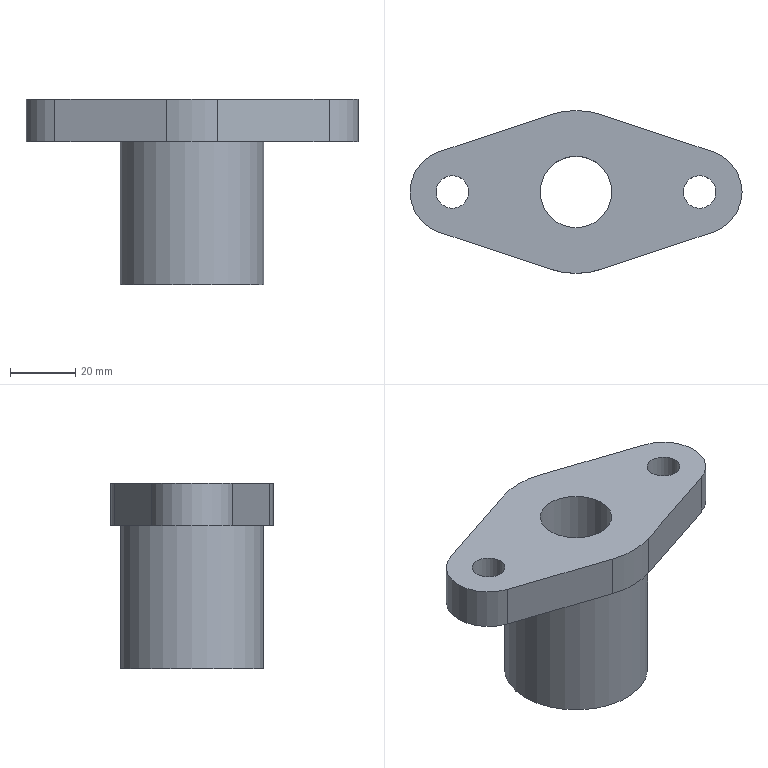Component | NX | 06__GLAND__2 | 1 solid | 15 faces | box 102 x 50 x 57 mm | volume 86309 mm3 | cylinder 8 | plane 6 | cone 1 | commonest cylinder face diameters 26 x2 50 x2 10 x2 22 x1 44 x1
STEP:
#1=CARTESIAN_POINT('',(0.,0.,0.));
#2=DIRECTION('',(0.,0.,1.));
#3=DIRECTION('',(1.,0.,0.));
#4=AXIS2_PLACEMENT_3D('',#1,#2,#3);
#5=CARTESIAN_POINT('',(35.73,-13.604,857.));
#6=VERTEX_POINT('',#5);
#7=CARTESIAN_POINT('',(35.73,11.065,857.));
#8=VERTEX_POINT('',#7);
#9=CARTESIAN_POINT('',(31.625,-1.269,857.));
#10=DIRECTION('',(0.,0.,1.));
#11=DIRECTION('',(-1.,-0.,0.));
#12=AXIS2_PLACEMENT_3D('',#9,#10,#11);
#13=CIRCLE('',#12,13.);
#14=CARTESIAN_POINT('',(31.625,-1.269,870.));
#15=DIRECTION('',(0.,0.,-1.));
#16=DIRECTION('',(1.,0.,0.));
#17=AXIS2_PLACEMENT_3D('',#14,#15,#16);
#18=CYLINDRICAL_SURFACE('',#17,13.);
#19=CARTESIAN_POINT('',(3.142,13.));
#20=DIRECTION('',(-1.,0.));
#21=VECTOR('',#20,1.);
#22=LINE('',#19,#21);
#23=(GEOMETRIC_REPRESENTATION_CONTEXT(2)PARAMETRIC_REPRESENTATION_CONTEXT()REPRESENTATION_CONTEXT('',''));
#24=DEFINITIONAL_REPRESENTATION('',(#22),#23);
#25=PCURVE('',#18,#24);
#26=CARTESIAN_POINT('',(31.625,-1.269,857.));
#27=DIRECTION('',(0.,0.,1.));
#28=DIRECTION('',(-1.,-0.,0.));
#29=AXIS2_PLACEMENT_3D('',#26,#27,#28);
#30=PLANE('',#29);
#31=CARTESIAN_POINT('',(0.,0.));
#32=DIRECTION('',(1.,0.));
#33=AXIS2_PLACEMENT_2D('',#31,#32);
#34=CIRCLE('',#33,13.);
#35=(GEOMETRIC_REPRESENTATION_CONTEXT(2)PARAMETRIC_REPRESENTATION_CONTEXT()REPRESENTATION_CONTEXT('',''));
#36=DEFINITIONAL_REPRESENTATION('',(#34),#35);
#37=PCURVE('',#30,#36);
#38=SURFACE_CURVE('',#13,(#25,#37),.PCURVE_S1.);
#39=EDGE_CURVE('',#6,#8,#38,.T.);
#40=ORIENTED_EDGE('',*,*,#39,.T.);
#41=CARTESIAN_POINT('',(35.73,11.065,870.));
#42=VERTEX_POINT('',#41);
#43=CARTESIAN_POINT('',(35.73,11.065,870.));
#44=DIRECTION('',(0.,0.,-1.));
#45=VECTOR('',#44,1.);
#46=LINE('',#43,#45);
#47=CARTESIAN_POINT('',(-1.25,0.));
#48=DIRECTION('',(0.,1.));
#49=VECTOR('',#48,1.);
#50=LINE('',#47,#49);
#51=(GEOMETRIC_REPRESENTATION_CONTEXT(2)PARAMETRIC_REPRESENTATION_CONTEXT()REPRESENTATION_CONTEXT('',''));
#52=DEFINITIONAL_REPRESENTATION('',(#50),#51);
#53=PCURVE('',#18,#52);
#54=CARTESIAN_POINT('',(35.73,11.065,870.));
#55=DIRECTION('',(-0.3158,-0.9488,0.));
#56=DIRECTION('',(0.9488,-0.3158,0.));
#57=AXIS2_PLACEMENT_3D('',#54,#55,#56);
#58=PLANE('',#57);
#59=CARTESIAN_POINT('',(-0.,0.));
#60=DIRECTION('',(0.,-1.));
#61=VECTOR('',#60,1.);
#62=LINE('',#59,#61);
#63=(GEOMETRIC_REPRESENTATION_CONTEXT(2)PARAMETRIC_REPRESENTATION_CONTEXT()REPRESENTATION_CONTEXT('',''));
#64=DEFINITIONAL_REPRESENTATION('',(#62),#63);
#65=PCURVE('',#58,#64);
#66=SURFACE_CURVE('',#46,(#53,#65),.PCURVE_S1.);
#67=EDGE_CURVE('',#42,#8,#66,.T.);
#68=ORIENTED_EDGE('',*,*,#67,.F.);
#69=CARTESIAN_POINT('',(35.73,-13.604,870.));
#70=VERTEX_POINT('',#69);
#71=CARTESIAN_POINT('',(31.625,-1.269,870.));
#72=DIRECTION('',(0.,0.,1.));
#73=DIRECTION('',(-1.,-0.,0.));
#74=AXIS2_PLACEMENT_3D('',#71,#72,#73);
#75=CIRCLE('',#74,13.);
#76=CARTESIAN_POINT('',(3.142,0.));
#77=DIRECTION('',(-1.,0.));
#78=VECTOR('',#77,1.);
#79=LINE('',#76,#78);
#80=(GEOMETRIC_REPRESENTATION_CONTEXT(2)PARAMETRIC_REPRESENTATION_CONTEXT()REPRESENTATION_CONTEXT('',''));
#81=DEFINITIONAL_REPRESENTATION('',(#79),#80);
#82=PCURVE('',#18,#81);
#83=CARTESIAN_POINT('',(31.625,-1.269,870.));
#84=DIRECTION('',(0.,0.,1.));
#85=DIRECTION('',(-1.,-0.,0.));
#86=AXIS2_PLACEMENT_3D('',#83,#84,#85);
#87=PLANE('',#86);
#88=CARTESIAN_POINT('',(0.,0.));
#89=DIRECTION('',(1.,0.));
#90=AXIS2_PLACEMENT_2D('',#88,#89);
#91=CIRCLE('',#90,13.);
#92=(GEOMETRIC_REPRESENTATION_CONTEXT(2)PARAMETRIC_REPRESENTATION_CONTEXT()REPRESENTATION_CONTEXT('',''));
#93=DEFINITIONAL_REPRESENTATION('',(#91),#92);
#94=PCURVE('',#87,#93);
#95=SURFACE_CURVE('',#75,(#82,#94),.PCURVE_S1.);
#96=EDGE_CURVE('',#70,#42,#95,.T.);
#97=ORIENTED_EDGE('',*,*,#96,.F.);
#98=CARTESIAN_POINT('',(35.73,-13.604,870.));
#99=DIRECTION('',(0.,0.,-1.));
#100=VECTOR('',#99,1.);
#101=LINE('',#98,#100);
#102=CARTESIAN_POINT('',(1.25,0.));
#103=DIRECTION('',(0.,1.));
#104=VECTOR('',#103,1.);
#105=LINE('',#102,#104);
#106=(GEOMETRIC_REPRESENTATION_CONTEXT(2)PARAMETRIC_REPRESENTATION_CONTEXT()REPRESENTATION_CONTEXT('',''));
#107=DEFINITIONAL_REPRESENTATION('',(#105),#106);
#108=PCURVE('',#18,#107);
#109=CARTESIAN_POINT('',(1.52,-24.99,870.));
#110=DIRECTION('',(-0.3158,0.9488,0.));
#111=DIRECTION('',(-0.9488,-0.3158,0.));
#112=AXIS2_PLACEMENT_3D('',#109,#110,#111);
#113=PLANE('',#112);
#114=CARTESIAN_POINT('',(-36.056,0.));
#115=DIRECTION('',(0.,-1.));
#116=VECTOR('',#115,1.);
#117=LINE('',#114,#116);
#118=(GEOMETRIC_REPRESENTATION_CONTEXT(2)PARAMETRIC_REPRESENTATION_CONTEXT()REPRESENTATION_CONTEXT('',''));
#119=DEFINITIONAL_REPRESENTATION('',(#117),#118);
#120=PCURVE('',#113,#119);
#121=SURFACE_CURVE('',#101,(#108,#120),.PCURVE_S1.);
#122=EDGE_CURVE('',#70,#6,#121,.T.);
#123=ORIENTED_EDGE('',*,*,#122,.T.);
#124=EDGE_LOOP('',(#40,#68,#97,#123));
#125=FACE_BOUND('',#124,.T.);
#126=ADVANCED_FACE('',(#125),#18,.T.);
#127=CARTESIAN_POINT('',(1.52,22.451,857.));
#128=VERTEX_POINT('',#127);
#129=CARTESIAN_POINT('',(35.73,11.065,857.));
#130=DIRECTION('',(-0.9488,0.3158,0.));
#131=VECTOR('',#130,1.);
#132=LINE('',#129,#131);
#133=CARTESIAN_POINT('',(0.,-13.));
#134=DIRECTION('',(-1.,0.));
#135=VECTOR('',#134,1.);
#136=LINE('',#133,#135);
#137=(GEOMETRIC_REPRESENTATION_CONTEXT(2)PARAMETRIC_REPRESENTATION_CONTEXT()REPRESENTATION_CONTEXT('',''));
#138=DEFINITIONAL_REPRESENTATION('',(#136),#137);
#139=PCURVE('',#58,#138);
#140=CARTESIAN_POINT('',(-4.105,-12.335));
#141=DIRECTION('',(0.9488,-0.3158));
#142=VECTOR('',#141,1.);
#143=LINE('',#140,#142);
#144=(GEOMETRIC_REPRESENTATION_CONTEXT(2)PARAMETRIC_REPRESENTATION_CONTEXT()REPRESENTATION_CONTEXT('',''));
#145=DEFINITIONAL_REPRESENTATION('',(#143),#144);
#146=PCURVE('',#30,#145);
#147=SURFACE_CURVE('',#132,(#139,#146),.PCURVE_S1.);
#148=EDGE_CURVE('',#8,#128,#147,.T.);
#149=ORIENTED_EDGE('',*,*,#148,.T.);
#150=CARTESIAN_POINT('',(1.52,22.451,870.));
#151=VERTEX_POINT('',#150);
#152=CARTESIAN_POINT('',(1.52,22.451,870.));
#153=DIRECTION('',(0.,0.,-1.));
#154=VECTOR('',#153,1.);
#155=LINE('',#152,#154);
#156=CARTESIAN_POINT('',(-36.056,0.));
#157=DIRECTION('',(0.,-1.));
#158=VECTOR('',#157,1.);
#159=LINE('',#156,#158);
#160=(GEOMETRIC_REPRESENTATION_CONTEXT(2)PARAMETRIC_REPRESENTATION_CONTEXT()REPRESENTATION_CONTEXT('',''));
#161=DEFINITIONAL_REPRESENTATION('',(#159),#160);
#162=PCURVE('',#58,#161);
#163=CARTESIAN_POINT('',(-6.375,-1.269,870.));
#164=DIRECTION('',(0.,0.,-1.));
#165=DIRECTION('',(1.,0.,0.));
#166=AXIS2_PLACEMENT_3D('',#163,#164,#165);
#167=CYLINDRICAL_SURFACE('',#166,25.);
#168=CARTESIAN_POINT('',(5.034,0.));
#169=DIRECTION('',(0.,1.));
#170=VECTOR('',#169,1.);
#171=LINE('',#168,#170);
#172=(GEOMETRIC_REPRESENTATION_CONTEXT(2)PARAMETRIC_REPRESENTATION_CONTEXT()REPRESENTATION_CONTEXT('',''));
#173=DEFINITIONAL_REPRESENTATION('',(#171),#172);
#174=PCURVE('',#167,#173);
#175=SURFACE_CURVE('',#155,(#162,#174),.PCURVE_S1.);
#176=EDGE_CURVE('',#151,#128,#175,.T.);
#177=ORIENTED_EDGE('',*,*,#176,.F.);
#178=CARTESIAN_POINT('',(35.73,11.065,870.));
#179=DIRECTION('',(-0.9488,0.3158,0.));
#180=VECTOR('',#179,1.);
#181=LINE('',#178,#180);
#182=CARTESIAN_POINT('',(0.,0.));
#183=DIRECTION('',(-1.,0.));
#184=VECTOR('',#183,1.);
#185=LINE('',#182,#184);
#186=(GEOMETRIC_REPRESENTATION_CONTEXT(2)PARAMETRIC_REPRESENTATION_CONTEXT()REPRESENTATION_CONTEXT('',''));
#187=DEFINITIONAL_REPRESENTATION('',(#185),#186);
#188=PCURVE('',#58,#187);
#189=CARTESIAN_POINT('',(-4.105,-12.335));
#190=DIRECTION('',(0.9488,-0.3158));
#191=VECTOR('',#190,1.);
#192=LINE('',#189,#191);
#193=(GEOMETRIC_REPRESENTATION_CONTEXT(2)PARAMETRIC_REPRESENTATION_CONTEXT()REPRESENTATION_CONTEXT('',''));
#194=DEFINITIONAL_REPRESENTATION('',(#192),#193);
#195=PCURVE('',#87,#194);
#196=SURFACE_CURVE('',#181,(#188,#195),.PCURVE_S1.);
#197=EDGE_CURVE('',#42,#151,#196,.T.);
#198=ORIENTED_EDGE('',*,*,#197,.F.);
#199=ORIENTED_EDGE('',*,*,#67,.T.);
#200=EDGE_LOOP('',(#149,#177,#198,#199));
#201=FACE_BOUND('',#200,.T.);
#202=ADVANCED_FACE('',(#201),#58,.F.);
#203=CARTESIAN_POINT('',(-14.27,22.451,857.));
#204=VERTEX_POINT('',#203);
#205=CARTESIAN_POINT('',(-6.375,-1.269,857.));
#206=DIRECTION('',(0.,0.,1.));
#207=DIRECTION('',(-1.,-0.,0.));
#208=AXIS2_PLACEMENT_3D('',#205,#206,#207);
#209=CIRCLE('',#208,25.);
#210=CARTESIAN_POINT('',(9.425,13.));
#211=DIRECTION('',(-1.,0.));
#212=VECTOR('',#211,1.);
#213=LINE('',#210,#212);
#214=(GEOMETRIC_REPRESENTATION_CONTEXT(2)PARAMETRIC_REPRESENTATION_CONTEXT()REPRESENTATION_CONTEXT('',''));
#215=DEFINITIONAL_REPRESENTATION('',(#213),#214);
#216=PCURVE('',#167,#215);
#217=CARTESIAN_POINT('',(38.,0.));
#218=DIRECTION('',(1.,-0.));
#219=AXIS2_PLACEMENT_2D('',#217,#218);
#220=CIRCLE('',#219,25.);
#221=(GEOMETRIC_REPRESENTATION_CONTEXT(2)PARAMETRIC_REPRESENTATION_CONTEXT()REPRESENTATION_CONTEXT('',''));
#222=DEFINITIONAL_REPRESENTATION('',(#220),#221);
#223=PCURVE('',#30,#222);
#224=SURFACE_CURVE('',#209,(#216,#223),.PCURVE_S1.);
#225=EDGE_CURVE('',#128,#204,#224,.T.);
#226=ORIENTED_EDGE('',*,*,#225,.T.);
#227=CARTESIAN_POINT('',(-14.27,22.451,870.));
#228=VERTEX_POINT('',#227);
#229=CARTESIAN_POINT('',(-14.27,22.451,870.));
#230=DIRECTION('',(0.,0.,-1.));
#231=VECTOR('',#230,1.);
#232=LINE('',#229,#231);
#233=CARTESIAN_POINT('',(4.391,0.));
#234=DIRECTION('',(0.,1.));
#235=VECTOR('',#234,1.);
#236=LINE('',#233,#235);
#237=(GEOMETRIC_REPRESENTATION_CONTEXT(2)PARAMETRIC_REPRESENTATION_CONTEXT()REPRESENTATION_CONTEXT('',''));
#238=DEFINITIONAL_REPRESENTATION('',(#236),#237);
#239=PCURVE('',#167,#238);
#240=CARTESIAN_POINT('',(-14.27,22.451,870.));
#241=DIRECTION('',(0.3158,-0.9488,0.));
#242=DIRECTION('',(0.9488,0.3158,0.));
#243=AXIS2_PLACEMENT_3D('',#240,#241,#242);
#244=PLANE('',#243);
#245=CARTESIAN_POINT('',(0.,0.));
#246=DIRECTION('',(0.,-1.));
#247=VECTOR('',#246,1.);
#248=LINE('',#245,#247);
#249=(GEOMETRIC_REPRESENTATION_CONTEXT(2)PARAMETRIC_REPRESENTATION_CONTEXT()REPRESENTATION_CONTEXT('',''));
#250=DEFINITIONAL_REPRESENTATION('',(#248),#249);
#251=PCURVE('',#244,#250);
#252=SURFACE_CURVE('',#232,(#239,#251),.PCURVE_S1.);
#253=EDGE_CURVE('',#228,#204,#252,.T.);
#254=ORIENTED_EDGE('',*,*,#253,.F.);
#255=CARTESIAN_POINT('',(-6.375,-1.269,870.));
#256=DIRECTION('',(0.,0.,1.));
#257=DIRECTION('',(-1.,-0.,0.));
#258=AXIS2_PLACEMENT_3D('',#255,#256,#257);
#259=CIRCLE('',#258,25.);
#260=CARTESIAN_POINT('',(9.425,0.));
#261=DIRECTION('',(-1.,0.));
#262=VECTOR('',#261,1.);
#263=LINE('',#260,#262);
#264=(GEOMETRIC_REPRESENTATION_CONTEXT(2)PARAMETRIC_REPRESENTATION_CONTEXT()REPRESENTATION_CONTEXT('',''));
#265=DEFINITIONAL_REPRESENTATION('',(#263),#264);
#266=PCURVE('',#167,#265);
#267=CARTESIAN_POINT('',(38.,0.));
#268=DIRECTION('',(1.,-0.));
#269=AXIS2_PLACEMENT_2D('',#267,#268);
#270=CIRCLE('',#269,25.);
#271=(GEOMETRIC_REPRESENTATION_CONTEXT(2)PARAMETRIC_REPRESENTATION_CONTEXT()REPRESENTATION_CONTEXT('',''));
#272=DEFINITIONAL_REPRESENTATION('',(#270),#271);
#273=PCURVE('',#87,#272);
#274=SURFACE_CURVE('',#259,(#266,#273),.PCURVE_S1.);
#275=EDGE_CURVE('',#151,#228,#274,.T.);
#276=ORIENTED_EDGE('',*,*,#275,.F.);
#277=ORIENTED_EDGE('',*,*,#176,.T.);
#278=EDGE_LOOP('',(#226,#254,#276,#277));
#279=FACE_BOUND('',#278,.T.);
#280=ADVANCED_FACE('',(#279),#167,.T.);
#281=CARTESIAN_POINT('',(-48.48,11.065,857.));
#282=VERTEX_POINT('',#281);
#283=CARTESIAN_POINT('',(-14.27,22.451,857.));
#284=DIRECTION('',(-0.9488,-0.3158,0.));
#285=VECTOR('',#284,1.);
#286=LINE('',#283,#285);
#287=CARTESIAN_POINT('',(0.,-13.));
#288=DIRECTION('',(-1.,0.));
#289=VECTOR('',#288,1.);
#290=LINE('',#287,#289);
#291=(GEOMETRIC_REPRESENTATION_CONTEXT(2)PARAMETRIC_REPRESENTATION_CONTEXT()REPRESENTATION_CONTEXT('',''));
#292=DEFINITIONAL_REPRESENTATION('',(#290),#291);
#293=PCURVE('',#244,#292);
#294=CARTESIAN_POINT('',(45.895,-23.721));
#295=DIRECTION('',(0.9488,0.3158));
#296=VECTOR('',#295,1.);
#297=LINE('',#294,#296);
#298=(GEOMETRIC_REPRESENTATION_CONTEXT(2)PARAMETRIC_REPRESENTATION_CONTEXT()REPRESENTATION_CONTEXT('',''));
#299=DEFINITIONAL_REPRESENTATION('',(#297),#298);
#300=PCURVE('',#30,#299);
#301=SURFACE_CURVE('',#286,(#293,#300),.PCURVE_S1.);
#302=EDGE_CURVE('',#204,#282,#301,.T.);
#303=ORIENTED_EDGE('',*,*,#302,.T.);
#304=CARTESIAN_POINT('',(-48.48,11.065,870.));
#305=VERTEX_POINT('',#304);
#306=CARTESIAN_POINT('',(-48.48,11.065,870.));
#307=DIRECTION('',(0.,0.,-1.));
#308=VECTOR('',#307,1.);
#309=LINE('',#306,#308);
#310=CARTESIAN_POINT('',(-36.056,0.));
#311=DIRECTION('',(0.,-1.));
#312=VECTOR('',#311,1.);
#313=LINE('',#310,#312);
#314=(GEOMETRIC_REPRESENTATION_CONTEXT(2)PARAMETRIC_REPRESENTATION_CONTEXT()REPRESENTATION_CONTEXT('',''));
#315=DEFINITIONAL_REPRESENTATION('',(#313),#314);
#316=PCURVE('',#244,#315);
#317=CARTESIAN_POINT('',(-44.375,-1.269,870.));
#318=DIRECTION('',(0.,0.,-1.));
#319=DIRECTION('',(1.,0.,0.));
#320=AXIS2_PLACEMENT_3D('',#317,#318,#319);
#321=CYLINDRICAL_SURFACE('',#320,13.);
#322=CARTESIAN_POINT('',(4.391,0.));
#323=DIRECTION('',(0.,1.));
#324=VECTOR('',#323,1.);
#325=LINE('',#322,#324);
#326=(GEOMETRIC_REPRESENTATION_CONTEXT(2)PARAMETRIC_REPRESENTATION_CONTEXT()REPRESENTATION_CONTEXT('',''));
#327=DEFINITIONAL_REPRESENTATION('',(#325),#326);
#328=PCURVE('',#321,#327);
#329=SURFACE_CURVE('',#309,(#316,#328),.PCURVE_S1.);
#330=EDGE_CURVE('',#305,#282,#329,.T.);
#331=ORIENTED_EDGE('',*,*,#330,.F.);
#332=CARTESIAN_POINT('',(-14.27,22.451,870.));
#333=DIRECTION('',(-0.9488,-0.3158,0.));
#334=VECTOR('',#333,1.);
#335=LINE('',#332,#334);
#336=CARTESIAN_POINT('',(0.,0.));
#337=DIRECTION('',(-1.,0.));
#338=VECTOR('',#337,1.);
#339=LINE('',#336,#338);
#340=(GEOMETRIC_REPRESENTATION_CONTEXT(2)PARAMETRIC_REPRESENTATION_CONTEXT()REPRESENTATION_CONTEXT('',''));
#341=DEFINITIONAL_REPRESENTATION('',(#339),#340);
#342=PCURVE('',#244,#341);
#343=CARTESIAN_POINT('',(45.895,-23.721));
#344=DIRECTION('',(0.9488,0.3158));
#345=VECTOR('',#344,1.);
#346=LINE('',#343,#345);
#347=(GEOMETRIC_REPRESENTATION_CONTEXT(2)PARAMETRIC_REPRESENTATION_CONTEXT()REPRESENTATION_CONTEXT('',''));
#348=DEFINITIONAL_REPRESENTATION('',(#346),#347);
#349=PCURVE('',#87,#348);
#350=SURFACE_CURVE('',#335,(#342,#349),.PCURVE_S1.);
#351=EDGE_CURVE('',#228,#305,#350,.T.);
#352=ORIENTED_EDGE('',*,*,#351,.F.);
#353=ORIENTED_EDGE('',*,*,#253,.T.);
#354=EDGE_LOOP('',(#303,#331,#352,#353));
#355=FACE_BOUND('',#354,.T.);
#356=ADVANCED_FACE('',(#355),#244,.F.);
#357=CARTESIAN_POINT('',(-48.48,-13.604,857.));
#358=VERTEX_POINT('',#357);
#359=CARTESIAN_POINT('',(-44.375,-1.269,857.));
#360=DIRECTION('',(0.,0.,1.));
#361=DIRECTION('',(1.,0.,0.));
#362=AXIS2_PLACEMENT_3D('',#359,#360,#361);
#363=CIRCLE('',#362,13.);
#364=CARTESIAN_POINT('',(6.283,13.));
#365=DIRECTION('',(-1.,0.));
#366=VECTOR('',#365,1.);
#367=LINE('',#364,#366);
#368=(GEOMETRIC_REPRESENTATION_CONTEXT(2)PARAMETRIC_REPRESENTATION_CONTEXT()REPRESENTATION_CONTEXT('',''));
#369=DEFINITIONAL_REPRESENTATION('',(#367),#368);
#370=PCURVE('',#321,#369);
#371=CARTESIAN_POINT('',(76.,0.));
#372=DIRECTION('',(-1.,0.));
#373=AXIS2_PLACEMENT_2D('',#371,#372);
#374=CIRCLE('',#373,13.);
#375=(GEOMETRIC_REPRESENTATION_CONTEXT(2)PARAMETRIC_REPRESENTATION_CONTEXT()REPRESENTATION_CONTEXT('',''));
#376=DEFINITIONAL_REPRESENTATION('',(#374),#375);
#377=PCURVE('',#30,#376);
#378=SURFACE_CURVE('',#363,(#370,#377),.PCURVE_S1.);
#379=EDGE_CURVE('',#282,#358,#378,.T.);
#380=ORIENTED_EDGE('',*,*,#379,.T.);
#381=CARTESIAN_POINT('',(-48.48,-13.604,870.));
#382=VERTEX_POINT('',#381);
#383=CARTESIAN_POINT('',(-48.48,-13.604,870.));
#384=DIRECTION('',(0.,0.,-1.));
#385=VECTOR('',#384,1.);
#386=LINE('',#383,#385);
#387=CARTESIAN_POINT('',(1.892,0.));
#388=DIRECTION('',(0.,1.));
#389=VECTOR('',#388,1.);
#390=LINE('',#387,#389);
#391=(GEOMETRIC_REPRESENTATION_CONTEXT(2)PARAMETRIC_REPRESENTATION_CONTEXT()REPRESENTATION_CONTEXT('',''));
#392=DEFINITIONAL_REPRESENTATION('',(#390),#391);
#393=PCURVE('',#321,#392);
#394=CARTESIAN_POINT('',(-48.48,-13.604,870.));
#395=DIRECTION('',(0.3158,0.9488,0.));
#396=DIRECTION('',(-0.9488,0.3158,0.));
#397=AXIS2_PLACEMENT_3D('',#394,#395,#396);
#398=PLANE('',#397);
#399=CARTESIAN_POINT('',(-0.,0.));
#400=DIRECTION('',(0.,-1.));
#401=VECTOR('',#400,1.);
#402=LINE('',#399,#401);
#403=(GEOMETRIC_REPRESENTATION_CONTEXT(2)PARAMETRIC_REPRESENTATION_CONTEXT()REPRESENTATION_CONTEXT('',''));
#404=DEFINITIONAL_REPRESENTATION('',(#402),#403);
#405=PCURVE('',#398,#404);
#406=SURFACE_CURVE('',#386,(#393,#405),.PCURVE_S1.);
#407=EDGE_CURVE('',#382,#358,#406,.T.);
#408=ORIENTED_EDGE('',*,*,#407,.F.);
#409=CARTESIAN_POINT('',(-44.375,-1.269,870.));
#410=DIRECTION('',(0.,0.,1.));
#411=DIRECTION('',(1.,0.,0.));
#412=AXIS2_PLACEMENT_3D('',#409,#410,#411);
#413=CIRCLE('',#412,13.);
#414=CARTESIAN_POINT('',(6.283,0.));
#415=DIRECTION('',(-1.,0.));
#416=VECTOR('',#415,1.);
#417=LINE('',#414,#416);
#418=(GEOMETRIC_REPRESENTATION_CONTEXT(2)PARAMETRIC_REPRESENTATION_CONTEXT()REPRESENTATION_CONTEXT('',''));
#419=DEFINITIONAL_REPRESENTATION('',(#417),#418);
#420=PCURVE('',#321,#419);
#421=CARTESIAN_POINT('',(76.,0.));
#422=DIRECTION('',(-1.,0.));
#423=AXIS2_PLACEMENT_2D('',#421,#422);
#424=CIRCLE('',#423,13.);
#425=(GEOMETRIC_REPRESENTATION_CONTEXT(2)PARAMETRIC_REPRESENTATION_CONTEXT()REPRESENTATION_CONTEXT('',''));
#426=DEFINITIONAL_REPRESENTATION('',(#424),#425);
#427=PCURVE('',#87,#426);
#428=SURFACE_CURVE('',#413,(#420,#427),.PCURVE_S1.);
#429=EDGE_CURVE('',#305,#382,#428,.T.);
#430=ORIENTED_EDGE('',*,*,#429,.F.);
#431=ORIENTED_EDGE('',*,*,#330,.T.);
#432=EDGE_LOOP('',(#380,#408,#430,#431));
#433=FACE_BOUND('',#432,.T.);
#434=ADVANCED_FACE('',(#433),#321,.T.);
#435=CARTESIAN_POINT('',(-14.27,-24.99,857.));
#436=VERTEX_POINT('',#435);
#437=CARTESIAN_POINT('',(-48.48,-13.604,857.));
#438=DIRECTION('',(0.9488,-0.3158,0.));
#439=VECTOR('',#438,1.);
#440=LINE('',#437,#439);
#441=CARTESIAN_POINT('',(0.,-13.));
#442=DIRECTION('',(-1.,0.));
#443=VECTOR('',#442,1.);
#444=LINE('',#441,#443);
#445=(GEOMETRIC_REPRESENTATION_CONTEXT(2)PARAMETRIC_REPRESENTATION_CONTEXT()REPRESENTATION_CONTEXT('',''));
#446=DEFINITIONAL_REPRESENTATION('',(#444),#445);
#447=PCURVE('',#398,#446);
#448=CARTESIAN_POINT('',(80.105,12.335));
#449=DIRECTION('',(-0.9488,0.3158));
#450=VECTOR('',#449,1.);
#451=LINE('',#448,#450);
#452=(GEOMETRIC_REPRESENTATION_CONTEXT(2)PARAMETRIC_REPRESENTATION_CONTEXT()REPRESENTATION_CONTEXT('',''));
#453=DEFINITIONAL_REPRESENTATION('',(#451),#452);
#454=PCURVE('',#30,#453);
#455=SURFACE_CURVE('',#440,(#447,#454),.PCURVE_S1.);
#456=EDGE_CURVE('',#358,#436,#455,.T.);
#457=ORIENTED_EDGE('',*,*,#456,.T.);
#458=CARTESIAN_POINT('',(-14.27,-24.99,870.));
#459=VERTEX_POINT('',#458);
#460=CARTESIAN_POINT('',(-14.27,-24.99,870.));
#461=DIRECTION('',(0.,0.,-1.));
#462=VECTOR('',#461,1.);
#463=LINE('',#460,#462);
#464=CARTESIAN_POINT('',(-36.056,0.));
#465=DIRECTION('',(0.,-1.));
#466=VECTOR('',#465,1.);
#467=LINE('',#464,#466);
#468=(GEOMETRIC_REPRESENTATION_CONTEXT(2)PARAMETRIC_REPRESENTATION_CONTEXT()REPRESENTATION_CONTEXT('',''));
#469=DEFINITIONAL_REPRESENTATION('',(#467),#468);
#470=PCURVE('',#398,#469);
#471=CARTESIAN_POINT('',(-6.375,-1.269,870.));
#472=DIRECTION('',(0.,0.,-1.));
#473=DIRECTION('',(1.,0.,0.));
#474=AXIS2_PLACEMENT_3D('',#471,#472,#473);
#475=CYLINDRICAL_SURFACE('',#474,25.);
#476=CARTESIAN_POINT('',(1.892,0.));
#477=DIRECTION('',(0.,1.));
#478=VECTOR('',#477,1.);
#479=LINE('',#476,#478);
#480=(GEOMETRIC_REPRESENTATION_CONTEXT(2)PARAMETRIC_REPRESENTATION_CONTEXT()REPRESENTATION_CONTEXT('',''));
#481=DEFINITIONAL_REPRESENTATION('',(#479),#480);
#482=PCURVE('',#475,#481);
#483=SURFACE_CURVE('',#463,(#470,#482),.PCURVE_S1.);
#484=EDGE_CURVE('',#459,#436,#483,.T.);
#485=ORIENTED_EDGE('',*,*,#484,.F.);
#486=CARTESIAN_POINT('',(-48.48,-13.604,870.));
#487=DIRECTION('',(0.9488,-0.3158,0.));
#488=VECTOR('',#487,1.);
#489=LINE('',#486,#488);
#490=CARTESIAN_POINT('',(0.,0.));
#491=DIRECTION('',(-1.,0.));
#492=VECTOR('',#491,1.);
#493=LINE('',#490,#492);
#494=(GEOMETRIC_REPRESENTATION_CONTEXT(2)PARAMETRIC_REPRESENTATION_CONTEXT()REPRESENTATION_CONTEXT('',''));
#495=DEFINITIONAL_REPRESENTATION('',(#493),#494);
#496=PCURVE('',#398,#495);
#497=CARTESIAN_POINT('',(80.105,12.335));
#498=DIRECTION('',(-0.9488,0.3158));
#499=VECTOR('',#498,1.);
#500=LINE('',#497,#499);
#501=(GEOMETRIC_REPRESENTATION_CONTEXT(2)PARAMETRIC_REPRESENTATION_CONTEXT()REPRESENTATION_CONTEXT('',''));
#502=DEFINITIONAL_REPRESENTATION('',(#500),#501);
#503=PCURVE('',#87,#502);
#504=SURFACE_CURVE('',#489,(#496,#503),.PCURVE_S1.);
#505=EDGE_CURVE('',#382,#459,#504,.T.);
#506=ORIENTED_EDGE('',*,*,#505,.F.);
#507=ORIENTED_EDGE('',*,*,#407,.T.);
#508=EDGE_LOOP('',(#457,#485,#506,#507));
#509=FACE_BOUND('',#508,.T.);
#510=ADVANCED_FACE('',(#509),#398,.F.);
#511=CARTESIAN_POINT('',(1.52,-24.99,857.));
#512=VERTEX_POINT('',#511);
#513=CARTESIAN_POINT('',(-6.375,-1.269,857.));
#514=DIRECTION('',(0.,0.,1.));
#515=DIRECTION('',(-1.,-0.,0.));
#516=AXIS2_PLACEMENT_3D('',#513,#514,#515);
#517=CIRCLE('',#516,25.);
#518=CARTESIAN_POINT('',(3.142,13.));
#519=DIRECTION('',(-1.,0.));
#520=VECTOR('',#519,1.);
#521=LINE('',#518,#520);
#522=(GEOMETRIC_REPRESENTATION_CONTEXT(2)PARAMETRIC_REPRESENTATION_CONTEXT()REPRESENTATION_CONTEXT('',''));
#523=DEFINITIONAL_REPRESENTATION('',(#521),#522);
#524=PCURVE('',#475,#523);
#525=CARTESIAN_POINT('',(38.,0.));
#526=DIRECTION('',(1.,-0.));
#527=AXIS2_PLACEMENT_2D('',#525,#526);
#528=CIRCLE('',#527,25.);
#529=(GEOMETRIC_REPRESENTATION_CONTEXT(2)PARAMETRIC_REPRESENTATION_CONTEXT()REPRESENTATION_CONTEXT('',''));
#530=DEFINITIONAL_REPRESENTATION('',(#528),#529);
#531=PCURVE('',#30,#530);
#532=SURFACE_CURVE('',#517,(#524,#531),.PCURVE_S1.);
#533=EDGE_CURVE('',#436,#512,#532,.T.);
#534=ORIENTED_EDGE('',*,*,#533,.T.);
#535=CARTESIAN_POINT('',(1.52,-24.99,870.));
#536=VERTEX_POINT('',#535);
#537=CARTESIAN_POINT('',(1.52,-24.99,870.));
#538=DIRECTION('',(0.,0.,-1.));
#539=VECTOR('',#538,1.);
#540=LINE('',#537,#539);
#541=CARTESIAN_POINT('',(1.25,0.));
#542=DIRECTION('',(0.,1.));
#543=VECTOR('',#542,1.);
#544=LINE('',#541,#543);
#545=(GEOMETRIC_REPRESENTATION_CONTEXT(2)PARAMETRIC_REPRESENTATION_CONTEXT()REPRESENTATION_CONTEXT('',''));
#546=DEFINITIONAL_REPRESENTATION('',(#544),#545);
#547=PCURVE('',#475,#546);
#548=CARTESIAN_POINT('',(0.,0.));
#549=DIRECTION('',(0.,-1.));
#550=VECTOR('',#549,1.);
#551=LINE('',#548,#550);
#552=(GEOMETRIC_REPRESENTATION_CONTEXT(2)PARAMETRIC_REPRESENTATION_CONTEXT()REPRESENTATION_CONTEXT('',''));
#553=DEFINITIONAL_REPRESENTATION('',(#551),#552);
#554=PCURVE('',#113,#553);
#555=SURFACE_CURVE('',#540,(#547,#554),.PCURVE_S1.);
#556=EDGE_CURVE('',#536,#512,#555,.T.);
#557=ORIENTED_EDGE('',*,*,#556,.F.);
#558=CARTESIAN_POINT('',(-6.375,-1.269,870.));
#559=DIRECTION('',(0.,0.,1.));
#560=DIRECTION('',(-1.,-0.,0.));
#561=AXIS2_PLACEMENT_3D('',#558,#559,#560);
#562=CIRCLE('',#561,25.);
#563=CARTESIAN_POINT('',(3.142,0.));
#564=DIRECTION('',(-1.,0.));
#565=VECTOR('',#564,1.);
#566=LINE('',#563,#565);
#567=(GEOMETRIC_REPRESENTATION_CONTEXT(2)PARAMETRIC_REPRESENTATION_CONTEXT()REPRESENTATION_CONTEXT('',''));
#568=DEFINITIONAL_REPRESENTATION('',(#566),#567);
#569=PCURVE('',#475,#568);
#570=CARTESIAN_POINT('',(38.,0.));
#571=DIRECTION('',(1.,-0.));
#572=AXIS2_PLACEMENT_2D('',#570,#571);
#573=CIRCLE('',#572,25.);
#574=(GEOMETRIC_REPRESENTATION_CONTEXT(2)PARAMETRIC_REPRESENTATION_CONTEXT()REPRESENTATION_CONTEXT('',''));
#575=DEFINITIONAL_REPRESENTATION('',(#573),#574);
#576=PCURVE('',#87,#575);
#577=SURFACE_CURVE('',#562,(#569,#576),.PCURVE_S1.);
#578=EDGE_CURVE('',#459,#536,#577,.T.);
#579=ORIENTED_EDGE('',*,*,#578,.F.);
#580=ORIENTED_EDGE('',*,*,#484,.T.);
#581=EDGE_LOOP('',(#534,#557,#579,#580));
#582=FACE_BOUND('',#581,.T.);
#583=ADVANCED_FACE('',(#582),#475,.T.);
#584=CARTESIAN_POINT('',(-17.375,-1.269,819.351));
#585=VERTEX_POINT('',#584);
#586=CARTESIAN_POINT('',(-6.375,-1.269,819.351));
#587=DIRECTION('',(0.,0.,-1.));
#588=DIRECTION('',(-1.,-0.,0.));
#589=AXIS2_PLACEMENT_3D('',#586,#587,#588);
#590=CIRCLE('',#589,11.);
#591=CARTESIAN_POINT('',(-6.375,-1.269,870.));
#592=DIRECTION('',(0.,0.,-1.));
#593=DIRECTION('',(1.,0.,0.));
#594=AXIS2_PLACEMENT_3D('',#591,#592,#593);
#595=CYLINDRICAL_SURFACE('',#594,11.);
#596=CARTESIAN_POINT('',(3.142,50.649));
#597=DIRECTION('',(1.,0.));
#598=VECTOR('',#597,1.);
#599=LINE('',#596,#598);
#600=(GEOMETRIC_REPRESENTATION_CONTEXT(2)PARAMETRIC_REPRESENTATION_CONTEXT()REPRESENTATION_CONTEXT('',''));
#601=DEFINITIONAL_REPRESENTATION('',(#599),#600);
#602=PCURVE('',#595,#601);
#603=CARTESIAN_POINT('',(-6.375,-1.269,813.));
#604=DIRECTION('',(0.,0.,-1.));
#605=DIRECTION('',(1.,0.,0.));
#606=AXIS2_PLACEMENT_3D('',#603,#604,#605);
#607=CONICAL_SURFACE('',#606,22.,1.047);
#608=CARTESIAN_POINT('',(3.142,-6.351));
#609=DIRECTION('',(1.,0.));
#610=VECTOR('',#609,1.);
#611=LINE('',#608,#610);
#612=(GEOMETRIC_REPRESENTATION_CONTEXT(2)PARAMETRIC_REPRESENTATION_CONTEXT()REPRESENTATION_CONTEXT('',''));
#613=DEFINITIONAL_REPRESENTATION('',(#611),#612);
#614=PCURVE('',#607,#613);
#615=SURFACE_CURVE('',#590,(#602,#614),.PCURVE_S1.);
#616=EDGE_CURVE('',#585,#585,#615,.T.);
#617=ORIENTED_EDGE('',*,*,#616,.F.);
#618=CARTESIAN_POINT('',(-17.375,-1.269,870.));
#619=VERTEX_POINT('',#618);
#620=CARTESIAN_POINT('',(-17.375,-1.269,870.));
#621=CARTESIAN_POINT('',(-17.375,-1.269,819.351));
#622=B_SPLINE_CURVE_WITH_KNOTS('',1,(#620,#621),.UNSPECIFIED.,.F.,.F.,(2,2),(0.,50.649),.PIECEWISE_BEZIER_KNOTS.);
#623=CARTESIAN_POINT('',(3.142,0.));
#624=DIRECTION('',(0.,1.));
#625=VECTOR('',#624,1.);
#626=LINE('',#623,#625);
#627=(GEOMETRIC_REPRESENTATION_CONTEXT(2)PARAMETRIC_REPRESENTATION_CONTEXT()REPRESENTATION_CONTEXT('',''));
#628=DEFINITIONAL_REPRESENTATION('',(#626),#627);
#629=PCURVE('',#595,#628);
#630=CARTESIAN_POINT('',(9.425,0.));
#631=DIRECTION('',(0.,1.));
#632=VECTOR('',#631,1.);
#633=LINE('',#630,#632);
#634=(GEOMETRIC_REPRESENTATION_CONTEXT(2)PARAMETRIC_REPRESENTATION_CONTEXT()REPRESENTATION_CONTEXT('',''));
#635=DEFINITIONAL_REPRESENTATION('',(#633),#634);
#636=PCURVE('',#595,#635);
#637=SEAM_CURVE('',#622,(#629,#636),.PCURVE_S1.);
#638=EDGE_CURVE('',#619,#585,#637,.T.);
#639=ORIENTED_EDGE('',*,*,#638,.F.);
#640=CARTESIAN_POINT('',(-6.375,-1.269,870.));
#641=DIRECTION('',(0.,0.,1.));
#642=DIRECTION('',(-1.,-0.,0.));
#643=AXIS2_PLACEMENT_3D('',#640,#641,#642);
#644=CIRCLE('',#643,11.);
#645=CARTESIAN_POINT('',(9.425,0.));
#646=DIRECTION('',(-1.,0.));
#647=VECTOR('',#646,1.);
#648=LINE('',#645,#647);
#649=(GEOMETRIC_REPRESENTATION_CONTEXT(2)PARAMETRIC_REPRESENTATION_CONTEXT()REPRESENTATION_CONTEXT('',''));
#650=DEFINITIONAL_REPRESENTATION('',(#648),#649);
#651=PCURVE('',#595,#650);
#652=CARTESIAN_POINT('',(38.,0.));
#653=DIRECTION('',(1.,-0.));
#654=AXIS2_PLACEMENT_2D('',#652,#653);
#655=CIRCLE('',#654,11.);
#656=(GEOMETRIC_REPRESENTATION_CONTEXT(2)PARAMETRIC_REPRESENTATION_CONTEXT()REPRESENTATION_CONTEXT('',''));
#657=DEFINITIONAL_REPRESENTATION('',(#655),#656);
#658=PCURVE('',#87,#657);
#659=SURFACE_CURVE('',#644,(#651,#658),.PCURVE_S1.);
#660=EDGE_CURVE('',#619,#619,#659,.T.);
#661=ORIENTED_EDGE('',*,*,#660,.F.);
#662=ORIENTED_EDGE('',*,*,#638,.T.);
#663=EDGE_LOOP('',(#617,#639,#661,#662));
#664=FACE_BOUND('',#663,.F.);
#665=ADVANCED_FACE('',(#664),#595,.F.);
#666=CARTESIAN_POINT('',(26.625,-1.269,870.));
#667=VERTEX_POINT('',#666);
#668=CARTESIAN_POINT('',(31.625,-1.269,870.));
#669=DIRECTION('',(0.,0.,1.));
#670=DIRECTION('',(-1.,-0.,0.));
#671=AXIS2_PLACEMENT_3D('',#668,#669,#670);
#672=CIRCLE('',#671,5.);
#673=CARTESIAN_POINT('',(31.625,-1.269,870.));
#674=DIRECTION('',(0.,0.,-1.));
#675=DIRECTION('',(1.,0.,0.));
#676=AXIS2_PLACEMENT_3D('',#673,#674,#675);
#677=CYLINDRICAL_SURFACE('',#676,5.);
#678=CARTESIAN_POINT('',(9.425,0.));
#679=DIRECTION('',(-1.,0.));
#680=VECTOR('',#679,1.);
#681=LINE('',#678,#680);
#682=(GEOMETRIC_REPRESENTATION_CONTEXT(2)PARAMETRIC_REPRESENTATION_CONTEXT()REPRESENTATION_CONTEXT('',''));
#683=DEFINITIONAL_REPRESENTATION('',(#681),#682);
#684=PCURVE('',#677,#683);
#685=CARTESIAN_POINT('',(0.,0.));
#686=DIRECTION('',(1.,-0.));
#687=AXIS2_PLACEMENT_2D('',#685,#686);
#688=CIRCLE('',#687,5.);
#689=(GEOMETRIC_REPRESENTATION_CONTEXT(2)PARAMETRIC_REPRESENTATION_CONTEXT()REPRESENTATION_CONTEXT('',''));
#690=DEFINITIONAL_REPRESENTATION('',(#688),#689);
#691=PCURVE('',#87,#690);
#692=SURFACE_CURVE('',#672,(#684,#691),.PCURVE_S1.);
#693=EDGE_CURVE('',#667,#667,#692,.T.);
#694=ORIENTED_EDGE('',*,*,#693,.F.);
#695=CARTESIAN_POINT('',(26.625,-1.269,857.));
#696=VERTEX_POINT('',#695);
#697=CARTESIAN_POINT('',(26.625,-1.269,870.));
#698=CARTESIAN_POINT('',(26.625,-1.269,857.));
#699=B_SPLINE_CURVE_WITH_KNOTS('',1,(#697,#698),.UNSPECIFIED.,.F.,.F.,(2,2),(0.,13.),.PIECEWISE_BEZIER_KNOTS.);
#700=CARTESIAN_POINT('',(9.425,0.));
#701=DIRECTION('',(0.,1.));
#702=VECTOR('',#701,1.);
#703=LINE('',#700,#702);
#704=(GEOMETRIC_REPRESENTATION_CONTEXT(2)PARAMETRIC_REPRESENTATION_CONTEXT()REPRESENTATION_CONTEXT('',''));
#705=DEFINITIONAL_REPRESENTATION('',(#703),#704);
#706=PCURVE('',#677,#705);
#707=CARTESIAN_POINT('',(3.142,0.));
#708=DIRECTION('',(0.,1.));
#709=VECTOR('',#708,1.);
#710=LINE('',#707,#709);
#711=(GEOMETRIC_REPRESENTATION_CONTEXT(2)PARAMETRIC_REPRESENTATION_CONTEXT()REPRESENTATION_CONTEXT('',''));
#712=DEFINITIONAL_REPRESENTATION('',(#710),#711);
#713=PCURVE('',#677,#712);
#714=SEAM_CURVE('',#699,(#706,#713),.PCURVE_S1.);
#715=EDGE_CURVE('',#667,#696,#714,.T.);
#716=ORIENTED_EDGE('',*,*,#715,.T.);
#717=CARTESIAN_POINT('',(31.625,-1.269,857.));
#718=DIRECTION('',(0.,0.,1.));
#719=DIRECTION('',(-1.,-0.,0.));
#720=AXIS2_PLACEMENT_3D('',#717,#718,#719);
#721=CIRCLE('',#720,5.);
#722=CARTESIAN_POINT('',(9.425,13.));
#723=DIRECTION('',(-1.,0.));
#724=VECTOR('',#723,1.);
#725=LINE('',#722,#724);
#726=(GEOMETRIC_REPRESENTATION_CONTEXT(2)PARAMETRIC_REPRESENTATION_CONTEXT()REPRESENTATION_CONTEXT('',''));
#727=DEFINITIONAL_REPRESENTATION('',(#725),#726);
#728=PCURVE('',#677,#727);
#729=CARTESIAN_POINT('',(0.,0.));
#730=DIRECTION('',(1.,-0.));
#731=AXIS2_PLACEMENT_2D('',#729,#730);
#732=CIRCLE('',#731,5.);
#733=(GEOMETRIC_REPRESENTATION_CONTEXT(2)PARAMETRIC_REPRESENTATION_CONTEXT()REPRESENTATION_CONTEXT('',''));
#734=DEFINITIONAL_REPRESENTATION('',(#732),#733);
#735=PCURVE('',#30,#734);
#736=SURFACE_CURVE('',#721,(#728,#735),.PCURVE_S1.);
#737=EDGE_CURVE('',#696,#696,#736,.T.);
#738=ORIENTED_EDGE('',*,*,#737,.T.);
#739=ORIENTED_EDGE('',*,*,#715,.F.);
#740=EDGE_LOOP('',(#694,#716,#738,#739));
#741=FACE_BOUND('',#740,.F.);
#742=ADVANCED_FACE('',(#741),#677,.F.);
#743=CARTESIAN_POINT('',(1.52,-24.99,857.));
#744=DIRECTION('',(0.9488,0.3158,0.));
#745=VECTOR('',#744,1.);
#746=LINE('',#743,#745);
#747=CARTESIAN_POINT('',(0.,-13.));
#748=DIRECTION('',(-1.,0.));
#749=VECTOR('',#748,1.);
#750=LINE('',#747,#749);
#751=(GEOMETRIC_REPRESENTATION_CONTEXT(2)PARAMETRIC_REPRESENTATION_CONTEXT()REPRESENTATION_CONTEXT('',''));
#752=DEFINITIONAL_REPRESENTATION('',(#750),#751);
#753=PCURVE('',#113,#752);
#754=CARTESIAN_POINT('',(30.105,23.721));
#755=DIRECTION('',(-0.9488,-0.3158));
#756=VECTOR('',#755,1.);
#757=LINE('',#754,#756);
#758=(GEOMETRIC_REPRESENTATION_CONTEXT(2)PARAMETRIC_REPRESENTATION_CONTEXT()REPRESENTATION_CONTEXT('',''));
#759=DEFINITIONAL_REPRESENTATION('',(#757),#758);
#760=PCURVE('',#30,#759);
#761=SURFACE_CURVE('',#746,(#753,#760),.PCURVE_S1.);
#762=EDGE_CURVE('',#512,#6,#761,.T.);
#763=ORIENTED_EDGE('',*,*,#762,.T.);
#764=ORIENTED_EDGE('',*,*,#122,.F.);
#765=CARTESIAN_POINT('',(1.52,-24.99,870.));
#766=DIRECTION('',(0.9488,0.3158,0.));
#767=VECTOR('',#766,1.);
#768=LINE('',#765,#767);
#769=CARTESIAN_POINT('',(0.,0.));
#770=DIRECTION('',(-1.,0.));
#771=VECTOR('',#770,1.);
#772=LINE('',#769,#771);
#773=(GEOMETRIC_REPRESENTATION_CONTEXT(2)PARAMETRIC_REPRESENTATION_CONTEXT()REPRESENTATION_CONTEXT('',''));
#774=DEFINITIONAL_REPRESENTATION('',(#772),#773);
#775=PCURVE('',#113,#774);
#776=CARTESIAN_POINT('',(30.105,23.721));
#777=DIRECTION('',(-0.9488,-0.3158));
#778=VECTOR('',#777,1.);
#779=LINE('',#776,#778);
#780=(GEOMETRIC_REPRESENTATION_CONTEXT(2)PARAMETRIC_REPRESENTATION_CONTEXT()REPRESENTATION_CONTEXT('',''));
#781=DEFINITIONAL_REPRESENTATION('',(#779),#780);
#782=PCURVE('',#87,#781);
#783=SURFACE_CURVE('',#768,(#775,#782),.PCURVE_S1.);
#784=EDGE_CURVE('',#536,#70,#783,.T.);
#785=ORIENTED_EDGE('',*,*,#784,.F.);
#786=ORIENTED_EDGE('',*,*,#556,.T.);
#787=EDGE_LOOP('',(#763,#764,#785,#786));
#788=FACE_BOUND('',#787,.T.);
#789=ADVANCED_FACE('',(#788),#113,.F.);
#790=CARTESIAN_POINT('',(-49.375,-1.269,870.));
#791=VERTEX_POINT('',#790);
#792=CARTESIAN_POINT('',(-44.375,-1.269,870.));
#793=DIRECTION('',(0.,0.,1.));
#794=DIRECTION('',(-1.,-0.,0.));
#795=AXIS2_PLACEMENT_3D('',#792,#793,#794);
#796=CIRCLE('',#795,5.);
#797=CARTESIAN_POINT('',(-44.375,-1.269,870.));
#798=DIRECTION('',(0.,0.,-1.));
#799=DIRECTION('',(1.,0.,0.));
#800=AXIS2_PLACEMENT_3D('',#797,#798,#799);
#801=CYLINDRICAL_SURFACE('',#800,5.);
#802=CARTESIAN_POINT('',(9.425,0.));
#803=DIRECTION('',(-1.,0.));
#804=VECTOR('',#803,1.);
#805=LINE('',#802,#804);
#806=(GEOMETRIC_REPRESENTATION_CONTEXT(2)PARAMETRIC_REPRESENTATION_CONTEXT()REPRESENTATION_CONTEXT('',''));
#807=DEFINITIONAL_REPRESENTATION('',(#805),#806);
#808=PCURVE('',#801,#807);
#809=CARTESIAN_POINT('',(76.,0.));
#810=DIRECTION('',(1.,-0.));
#811=AXIS2_PLACEMENT_2D('',#809,#810);
#812=CIRCLE('',#811,5.);
#813=(GEOMETRIC_REPRESENTATION_CONTEXT(2)PARAMETRIC_REPRESENTATION_CONTEXT()REPRESENTATION_CONTEXT('',''));
#814=DEFINITIONAL_REPRESENTATION('',(#812),#813);
#815=PCURVE('',#87,#814);
#816=SURFACE_CURVE('',#796,(#808,#815),.PCURVE_S1.);
#817=EDGE_CURVE('',#791,#791,#816,.T.);
#818=ORIENTED_EDGE('',*,*,#817,.F.);
#819=CARTESIAN_POINT('',(-49.375,-1.269,857.));
#820=VERTEX_POINT('',#819);
#821=CARTESIAN_POINT('',(-49.375,-1.269,870.));
#822=CARTESIAN_POINT('',(-49.375,-1.269,857.));
#823=B_SPLINE_CURVE_WITH_KNOTS('',1,(#821,#822),.UNSPECIFIED.,.F.,.F.,(2,2),(0.,13.),.PIECEWISE_BEZIER_KNOTS.);
#824=CARTESIAN_POINT('',(9.425,0.));
#825=DIRECTION('',(0.,1.));
#826=VECTOR('',#825,1.);
#827=LINE('',#824,#826);
#828=(GEOMETRIC_REPRESENTATION_CONTEXT(2)PARAMETRIC_REPRESENTATION_CONTEXT()REPRESENTATION_CONTEXT('',''));
#829=DEFINITIONAL_REPRESENTATION('',(#827),#828);
#830=PCURVE('',#801,#829);
#831=CARTESIAN_POINT('',(3.142,0.));
#832=DIRECTION('',(0.,1.));
#833=VECTOR('',#832,1.);
#834=LINE('',#831,#833);
#835=(GEOMETRIC_REPRESENTATION_CONTEXT(2)PARAMETRIC_REPRESENTATION_CONTEXT()REPRESENTATION_CONTEXT('',''));
#836=DEFINITIONAL_REPRESENTATION('',(#834),#835);
#837=PCURVE('',#801,#836);
#838=SEAM_CURVE('',#823,(#830,#837),.PCURVE_S1.);
#839=EDGE_CURVE('',#791,#820,#838,.T.);
#840=ORIENTED_EDGE('',*,*,#839,.T.);
#841=CARTESIAN_POINT('',(-44.375,-1.269,857.));
#842=DIRECTION('',(0.,0.,1.));
#843=DIRECTION('',(-1.,-0.,0.));
#844=AXIS2_PLACEMENT_3D('',#841,#842,#843);
#845=CIRCLE('',#844,5.);
#846=CARTESIAN_POINT('',(9.425,13.));
#847=DIRECTION('',(-1.,0.));
#848=VECTOR('',#847,1.);
#849=LINE('',#846,#848);
#850=(GEOMETRIC_REPRESENTATION_CONTEXT(2)PARAMETRIC_REPRESENTATION_CONTEXT()REPRESENTATION_CONTEXT('',''));
#851=DEFINITIONAL_REPRESENTATION('',(#849),#850);
#852=PCURVE('',#801,#851);
#853=CARTESIAN_POINT('',(76.,0.));
#854=DIRECTION('',(1.,-0.));
#855=AXIS2_PLACEMENT_2D('',#853,#854);
#856=CIRCLE('',#855,5.);
#857=(GEOMETRIC_REPRESENTATION_CONTEXT(2)PARAMETRIC_REPRESENTATION_CONTEXT()REPRESENTATION_CONTEXT('',''));
#858=DEFINITIONAL_REPRESENTATION('',(#856),#857);
#859=PCURVE('',#30,#858);
#860=SURFACE_CURVE('',#845,(#852,#859),.PCURVE_S1.);
#861=EDGE_CURVE('',#820,#820,#860,.T.);
#862=ORIENTED_EDGE('',*,*,#861,.T.);
#863=ORIENTED_EDGE('',*,*,#839,.F.);
#864=EDGE_LOOP('',(#818,#840,#862,#863));
#865=FACE_BOUND('',#864,.F.);
#866=ADVANCED_FACE('',(#865),#801,.F.);
#867=ORIENTED_EDGE('',*,*,#96,.T.);
#868=ORIENTED_EDGE('',*,*,#197,.T.);
#869=ORIENTED_EDGE('',*,*,#275,.T.);
#870=ORIENTED_EDGE('',*,*,#351,.T.);
#871=ORIENTED_EDGE('',*,*,#429,.T.);
#872=ORIENTED_EDGE('',*,*,#505,.T.);
#873=ORIENTED_EDGE('',*,*,#578,.T.);
#874=ORIENTED_EDGE('',*,*,#784,.T.);
#875=EDGE_LOOP('',(#867,#868,#869,#870,#871,#872,#873,#874));
#876=FACE_BOUND('',#875,.T.);
#877=ORIENTED_EDGE('',*,*,#693,.F.);
#878=EDGE_LOOP('',(#877));
#879=FACE_BOUND('',#878,.T.);
#880=ORIENTED_EDGE('',*,*,#660,.F.);
#881=EDGE_LOOP('',(#880));
#882=FACE_BOUND('',#881,.T.);
#883=ORIENTED_EDGE('',*,*,#817,.F.);
#884=EDGE_LOOP('',(#883));
#885=FACE_BOUND('',#884,.T.);
#886=ADVANCED_FACE('',(#876,#879,#882,#885),#87,.T.);
#887=CARTESIAN_POINT('',(-28.375,-1.269,857.));
#888=VERTEX_POINT('',#887);
#889=CARTESIAN_POINT('',(-6.375,-1.269,857.));
#890=DIRECTION('',(0.,0.,1.));
#891=DIRECTION('',(-1.,-0.,0.));
#892=AXIS2_PLACEMENT_3D('',#889,#890,#891);
#893=CIRCLE('',#892,22.);
#894=CARTESIAN_POINT('',(38.,0.));
#895=DIRECTION('',(1.,-0.));
#896=AXIS2_PLACEMENT_2D('',#894,#895);
#897=CIRCLE('',#896,22.);
#898=(GEOMETRIC_REPRESENTATION_CONTEXT(2)PARAMETRIC_REPRESENTATION_CONTEXT()REPRESENTATION_CONTEXT('',''));
#899=DEFINITIONAL_REPRESENTATION('',(#897),#898);
#900=PCURVE('',#30,#899);
#901=CARTESIAN_POINT('',(-6.375,-1.269,813.));
#902=DIRECTION('',(0.,0.,1.));
#903=DIRECTION('',(-1.,-0.,0.));
#904=AXIS2_PLACEMENT_3D('',#901,#902,#903);
#905=CYLINDRICAL_SURFACE('',#904,22.);
#906=CARTESIAN_POINT('',(0.,44.));
#907=DIRECTION('',(1.,0.));
#908=VECTOR('',#907,1.);
#909=LINE('',#906,#908);
#910=(GEOMETRIC_REPRESENTATION_CONTEXT(2)PARAMETRIC_REPRESENTATION_CONTEXT()REPRESENTATION_CONTEXT('',''));
#911=DEFINITIONAL_REPRESENTATION('',(#909),#910);
#912=PCURVE('',#905,#911);
#913=SURFACE_CURVE('',#893,(#900,#912),.PCURVE_S1.);
#914=EDGE_CURVE('',#888,#888,#913,.T.);
#915=ORIENTED_EDGE('',*,*,#914,.T.);
#916=EDGE_LOOP('',(#915));
#917=FACE_BOUND('',#916,.T.);
#918=ORIENTED_EDGE('',*,*,#39,.F.);
#919=ORIENTED_EDGE('',*,*,#762,.F.);
#920=ORIENTED_EDGE('',*,*,#533,.F.);
#921=ORIENTED_EDGE('',*,*,#456,.F.);
#922=ORIENTED_EDGE('',*,*,#379,.F.);
#923=ORIENTED_EDGE('',*,*,#302,.F.);
#924=ORIENTED_EDGE('',*,*,#225,.F.);
#925=ORIENTED_EDGE('',*,*,#148,.F.);
#926=EDGE_LOOP('',(#918,#919,#920,#921,#922,#923,#924,#925));
#927=FACE_BOUND('',#926,.T.);
#928=ORIENTED_EDGE('',*,*,#737,.T.);
#929=EDGE_LOOP('',(#928));
#930=FACE_BOUND('',#929,.T.);
#931=ORIENTED_EDGE('',*,*,#861,.T.);
#932=EDGE_LOOP('',(#931));
#933=FACE_BOUND('',#932,.T.);
#934=ADVANCED_FACE('',(#917,#927,#930,#933),#30,.F.);
#935=CARTESIAN_POINT('',(-28.375,-1.269,813.));
#936=VERTEX_POINT('',#935);
#937=CARTESIAN_POINT('',(-6.375,-1.269,813.));
#938=DIRECTION('',(0.,0.,1.));
#939=DIRECTION('',(-1.,-0.,0.));
#940=AXIS2_PLACEMENT_3D('',#937,#938,#939);
#941=CIRCLE('',#940,22.);
#942=CARTESIAN_POINT('',(0.,0.));
#943=DIRECTION('',(1.,0.));
#944=VECTOR('',#943,1.);
#945=LINE('',#942,#944);
#946=(GEOMETRIC_REPRESENTATION_CONTEXT(2)PARAMETRIC_REPRESENTATION_CONTEXT()REPRESENTATION_CONTEXT('',''));
#947=DEFINITIONAL_REPRESENTATION('',(#945),#946);
#948=PCURVE('',#905,#947);
#949=CARTESIAN_POINT('',(9.425,0.));
#950=DIRECTION('',(-1.,0.));
#951=VECTOR('',#950,1.);
#952=LINE('',#949,#951);
#953=(GEOMETRIC_REPRESENTATION_CONTEXT(2)PARAMETRIC_REPRESENTATION_CONTEXT()REPRESENTATION_CONTEXT('',''));
#954=DEFINITIONAL_REPRESENTATION('',(#952),#953);
#955=PCURVE('',#607,#954);
#956=SURFACE_CURVE('',#941,(#948,#955),.PCURVE_S1.);
#957=EDGE_CURVE('',#936,#936,#956,.T.);
#958=ORIENTED_EDGE('',*,*,#957,.T.);
#959=CARTESIAN_POINT('',(-28.375,-1.269,813.));
#960=CARTESIAN_POINT('',(-28.375,-1.269,857.));
#961=B_SPLINE_CURVE_WITH_KNOTS('',1,(#959,#960),.UNSPECIFIED.,.F.,.F.,(2,2),(0.,44.),.PIECEWISE_BEZIER_KNOTS.);
#962=CARTESIAN_POINT('',(6.283,0.));
#963=DIRECTION('',(0.,1.));
#964=VECTOR('',#963,1.);
#965=LINE('',#962,#964);
#966=(GEOMETRIC_REPRESENTATION_CONTEXT(2)PARAMETRIC_REPRESENTATION_CONTEXT()REPRESENTATION_CONTEXT('',''));
#967=DEFINITIONAL_REPRESENTATION('',(#965),#966);
#968=PCURVE('',#905,#967);
#969=CARTESIAN_POINT('',(0.,0.));
#970=DIRECTION('',(0.,1.));
#971=VECTOR('',#970,1.);
#972=LINE('',#969,#971);
#973=(GEOMETRIC_REPRESENTATION_CONTEXT(2)PARAMETRIC_REPRESENTATION_CONTEXT()REPRESENTATION_CONTEXT('',''));
#974=DEFINITIONAL_REPRESENTATION('',(#972),#973);
#975=PCURVE('',#905,#974);
#976=SEAM_CURVE('',#961,(#968,#975),.PCURVE_S1.);
#977=EDGE_CURVE('',#936,#888,#976,.T.);
#978=ORIENTED_EDGE('',*,*,#977,.T.);
#979=ORIENTED_EDGE('',*,*,#914,.F.);
#980=ORIENTED_EDGE('',*,*,#977,.F.);
#981=EDGE_LOOP('',(#958,#978,#979,#980));
#982=FACE_BOUND('',#981,.T.);
#983=ADVANCED_FACE('',(#982),#905,.T.);
#984=ORIENTED_EDGE('',*,*,#616,.T.);
#985=CARTESIAN_POINT('',(-17.375,-1.269,819.351));
#986=CARTESIAN_POINT('',(-28.375,-1.269,813.));
#987=B_SPLINE_CURVE_WITH_KNOTS('',1,(#985,#986),.UNSPECIFIED.,.F.,.F.,(2,2),(-12.702,0.),.PIECEWISE_BEZIER_KNOTS.);
#988=CARTESIAN_POINT('',(9.425,0.));
#989=DIRECTION('',(0.,1.));
#990=VECTOR('',#989,1.);
#991=LINE('',#988,#990);
#992=(GEOMETRIC_REPRESENTATION_CONTEXT(2)PARAMETRIC_REPRESENTATION_CONTEXT()REPRESENTATION_CONTEXT('',''));
#993=DEFINITIONAL_REPRESENTATION('',(#991),#992);
#994=PCURVE('',#607,#993);
#995=CARTESIAN_POINT('',(3.142,0.));
#996=DIRECTION('',(0.,1.));
#997=VECTOR('',#996,1.);
#998=LINE('',#995,#997);
#999=(GEOMETRIC_REPRESENTATION_CONTEXT(2)PARAMETRIC_REPRESENTATION_CONTEXT()REPRESENTATION_CONTEXT('',''));
#1000=DEFINITIONAL_REPRESENTATION('',(#998),#999);
#1001=PCURVE('',#607,#1000);
#1002=SEAM_CURVE('',#987,(#994,#1001),.PCURVE_S1.);
#1003=EDGE_CURVE('',#585,#936,#1002,.T.);
#1004=ORIENTED_EDGE('',*,*,#1003,.T.);
#1005=ORIENTED_EDGE('',*,*,#957,.T.);
#1006=ORIENTED_EDGE('',*,*,#1003,.F.);
#1007=EDGE_LOOP('',(#984,#1004,#1005,#1006));
#1008=FACE_BOUND('',#1007,.F.);
#1009=ADVANCED_FACE('',(#1008),#607,.F.);
#1010=CLOSED_SHELL('',(#126,#202,#280,#356,#434,#510,#583,#665,#742,#789,#866,#886,#934,#983,#1009));
#1011=MANIFOLD_SOLID_BREP('',#1010);
#1012=(LENGTH_UNIT()NAMED_UNIT(*)SI_UNIT(.MILLI.,.METRE.));
#1013=UNCERTAINTY_MEASURE_WITH_UNIT(LENGTH_MEASURE(0.000002),#1012,'','');
#1014=(NAMED_UNIT(*)PLANE_ANGLE_UNIT()SI_UNIT($,.RADIAN.));
#1015=(NAMED_UNIT(*)SI_UNIT($,.STERADIAN.)SOLID_ANGLE_UNIT());
#1016=(GEOMETRIC_REPRESENTATION_CONTEXT(3)GLOBAL_UNCERTAINTY_ASSIGNED_CONTEXT((#1013))GLOBAL_UNIT_ASSIGNED_CONTEXT((#1012,#1014,#1015))REPRESENTATION_CONTEXT('',''));
#1017=ADVANCED_BREP_SHAPE_REPRESENTATION('',(#4,#1011),#1016);